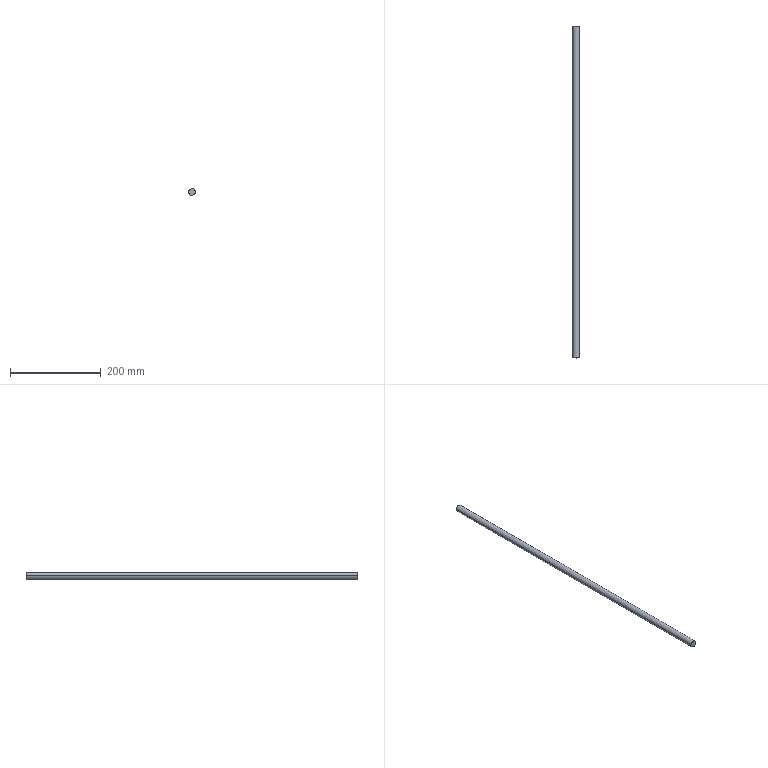Component | SolidWorks | InsectTrapLamp-1_BracketRod-5 | 1 solid | 4 faces | box 15 x 730 x 15 mm | volume 129002 mm3 | cylinder 2 | plane 2 | commonest cylinder face diameters 15 x2
build123d program:
from build123d import *

# Parameters (mm, degrees)
SKETCH1_R           = 7.5
BOSS_EXTRUDE1_DEPTH = 730


with BuildPart() as part:
    # Sketch1 → Boss-Extrude1 (new body)
    with BuildSketch(Plane(origin=(0, 0, 0), x_dir=(1, 0, 0), z_dir=(0, 1, 0))):
        with Locations(Location((0, 0, 0), (0, 0, 90))):
            Circle(SKETCH1_R)
    extrude(amount=BOSS_EXTRUDE1_DEPTH)


solid = part.part

# Placed as in the assembly
solid = solid.moved(Location((-155, 860, 155), (0, 0, 0)))
STEP:
#1=COLOUR_RGB('',0.7922,0.8196,0.9333);
#2=FILL_AREA_STYLE_COLOUR('',#1);
#3=FILL_AREA_STYLE('',(#2));
#4=SURFACE_STYLE_FILL_AREA(#3);
#5=SURFACE_SIDE_STYLE('',(#4));
#6=SURFACE_STYLE_USAGE(.BOTH.,#5);
#7=PRESENTATION_STYLE_ASSIGNMENT((#6));
#8=CARTESIAN_POINT('',(-6.396,62.598,6.132));
#9=VERTEX_POINT('',#8);
#10=CARTESIAN_POINT('',(-5.809,62.598,6.073));
#11=VERTEX_POINT('',#10);
#12=CARTESIAN_POINT('',(-6.102,62.598,6.102));
#13=DIRECTION('',(0.,1.,0.));
#14=DIRECTION('',(-0.9951,0.,0.0988));
#15=AXIS2_PLACEMENT_3D('',#12,#13,#14);
#16=CIRCLE('',#15,0.2953);
#17=EDGE_CURVE('',#9,#11,#16,.T.);
#18=ORIENTED_EDGE('',*,*,#17,.F.);
#19=CARTESIAN_POINT('',(-6.396,33.858,6.132));
#20=VERTEX_POINT('',#19);
#21=CARTESIAN_POINT('',(-6.396,62.598,6.132));
#22=DIRECTION('',(0.,-1.,0.));
#23=VECTOR('',#22,39.37);
#24=LINE('',#21,#23);
#25=EDGE_CURVE('',#9,#20,#24,.T.);
#26=ORIENTED_EDGE('',*,*,#25,.T.);
#27=CARTESIAN_POINT('',(-5.809,33.858,6.073));
#28=VERTEX_POINT('',#27);
#29=CARTESIAN_POINT('',(-6.102,33.858,6.102));
#30=DIRECTION('',(0.,1.,0.));
#31=DIRECTION('',(-0.9951,0.,0.0988));
#32=AXIS2_PLACEMENT_3D('',#29,#30,#31);
#33=CIRCLE('',#32,0.2953);
#34=EDGE_CURVE('',#20,#28,#33,.T.);
#35=ORIENTED_EDGE('',*,*,#34,.T.);
#36=CARTESIAN_POINT('',(-5.809,62.598,6.073));
#37=DIRECTION('',(0.,-1.,0.));
#38=VECTOR('',#37,39.37);
#39=LINE('',#36,#38);
#40=EDGE_CURVE('',#11,#28,#39,.T.);
#41=ORIENTED_EDGE('',*,*,#40,.F.);
#42=EDGE_LOOP('',(#18,#26,#35,#41));
#43=FACE_OUTER_BOUND('',#42,.T.);
#44=CARTESIAN_POINT('',(-6.102,62.598,6.102));
#45=DIRECTION('',(0.,-1.,0.));
#46=DIRECTION('',(0.9951,0.,-0.0988));
#47=AXIS2_PLACEMENT_3D('',#44,#45,#46);
#48=CYLINDRICAL_SURFACE('',#47,0.2953);
#49=ADVANCED_FACE('',(#43),#48,.T.);
#50=ORIENTED_EDGE('',*,*,#25,.F.);
#51=CARTESIAN_POINT('',(-6.102,62.598,6.102));
#52=DIRECTION('',(0.,1.,0.));
#53=DIRECTION('',(-0.9951,0.,0.0988));
#54=AXIS2_PLACEMENT_3D('',#51,#52,#53);
#55=CIRCLE('',#54,0.2953);
#56=EDGE_CURVE('',#11,#9,#55,.T.);
#57=ORIENTED_EDGE('',*,*,#56,.F.);
#58=ORIENTED_EDGE('',*,*,#40,.T.);
#59=CARTESIAN_POINT('',(-6.102,33.858,6.102));
#60=DIRECTION('',(0.,1.,0.));
#61=DIRECTION('',(-0.9951,0.,0.0988));
#62=AXIS2_PLACEMENT_3D('',#59,#60,#61);
#63=CIRCLE('',#62,0.2953);
#64=EDGE_CURVE('',#28,#20,#63,.T.);
#65=ORIENTED_EDGE('',*,*,#64,.T.);
#66=EDGE_LOOP('',(#50,#57,#58,#65));
#67=FACE_OUTER_BOUND('',#66,.T.);
#68=CARTESIAN_POINT('',(-6.102,62.598,6.102));
#69=DIRECTION('',(0.,-1.,0.));
#70=DIRECTION('',(0.9951,0.,-0.0988));
#71=AXIS2_PLACEMENT_3D('',#68,#69,#70);
#72=CYLINDRICAL_SURFACE('',#71,0.2953);
#73=ADVANCED_FACE('',(#67),#72,.T.);
#74=ORIENTED_EDGE('',*,*,#56,.T.);
#75=ORIENTED_EDGE('',*,*,#17,.T.);
#76=EDGE_LOOP('',(#74,#75));
#77=FACE_OUTER_BOUND('',#76,.T.);
#78=CARTESIAN_POINT('',(-6.102,62.598,6.102));
#79=DIRECTION('',(0.,1.,0.));
#80=DIRECTION('',(-0.9951,0.,0.0988));
#81=AXIS2_PLACEMENT_3D('',#78,#79,#80);
#82=PLANE('',#81);
#83=ADVANCED_FACE('',(#77),#82,.T.);
#84=ORIENTED_EDGE('',*,*,#64,.F.);
#85=ORIENTED_EDGE('',*,*,#34,.F.);
#86=EDGE_LOOP('',(#84,#85));
#87=FACE_OUTER_BOUND('',#86,.T.);
#88=CARTESIAN_POINT('',(-6.102,33.858,6.102));
#89=DIRECTION('',(0.,1.,0.));
#90=DIRECTION('',(-0.9951,0.,0.0988));
#91=AXIS2_PLACEMENT_3D('',#88,#89,#90);
#92=PLANE('',#91);
#93=ADVANCED_FACE('',(#87),#92,.F.);
#94=CLOSED_SHELL('',(#49,#73,#83,#93));
#95=MANIFOLD_SOLID_BREP('',#94);
#96=STYLED_ITEM('',(#7),#95);
#97=PRESENTATION_LAYER_ASSIGNMENT('','',(#96));
#98=(LENGTH_UNIT()NAMED_UNIT(*)SI_UNIT($,.METRE.));
#99=LENGTH_MEASURE_WITH_UNIT(LENGTH_MEASURE(0.0254),#98);
#100=DIMENSIONAL_EXPONENTS(1.,0.,0.,0.,0.,0.,0.);
#101=(CONVERSION_BASED_UNIT('',#99)LENGTH_UNIT()NAMED_UNIT(#100));
#102=UNCERTAINTY_MEASURE_WITH_UNIT(LENGTH_MEASURE(0.00001),#101,'','');
#103=(NAMED_UNIT(*)PLANE_ANGLE_UNIT()SI_UNIT($,.RADIAN.));
#104=(NAMED_UNIT(*)SI_UNIT($,.STERADIAN.)SOLID_ANGLE_UNIT());
#105=(GEOMETRIC_REPRESENTATION_CONTEXT(3)GLOBAL_UNCERTAINTY_ASSIGNED_CONTEXT((#102))GLOBAL_UNIT_ASSIGNED_CONTEXT((#101,#103,#104))REPRESENTATION_CONTEXT('',''));
#106=MECHANICAL_DESIGN_GEOMETRIC_PRESENTATION_REPRESENTATION('',(#96),#105);
#107=CARTESIAN_POINT('',(0.,0.,0.));
#108=DIRECTION('',(0.,0.,1.));
#109=DIRECTION('',(1.,0.,0.));
#110=AXIS2_PLACEMENT_3D('',#107,#108,#109);
#111=(LENGTH_UNIT()NAMED_UNIT(*)SI_UNIT($,.METRE.));
#112=LENGTH_MEASURE_WITH_UNIT(LENGTH_MEASURE(0.0254),#111);
#113=DIMENSIONAL_EXPONENTS(1.,0.,0.,0.,0.,0.,0.);
#114=(CONVERSION_BASED_UNIT('',#112)LENGTH_UNIT()NAMED_UNIT(#113));
#115=UNCERTAINTY_MEASURE_WITH_UNIT(LENGTH_MEASURE(0.00001),#114,'','');
#116=(NAMED_UNIT(*)PLANE_ANGLE_UNIT()SI_UNIT($,.RADIAN.));
#117=(NAMED_UNIT(*)SI_UNIT($,.STERADIAN.)SOLID_ANGLE_UNIT());
#118=(GEOMETRIC_REPRESENTATION_CONTEXT(3)GLOBAL_UNCERTAINTY_ASSIGNED_CONTEXT((#115))GLOBAL_UNIT_ASSIGNED_CONTEXT((#114,#116,#117))REPRESENTATION_CONTEXT('',''));
#119=ADVANCED_BREP_SHAPE_REPRESENTATION('',(#95,#110),#118);